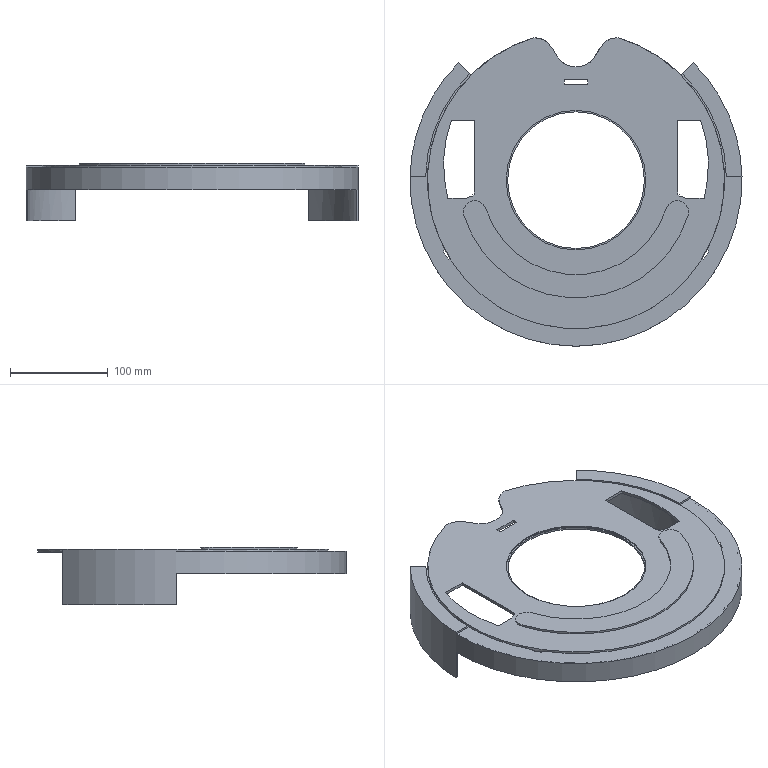Component | NX | OUTER_SHELL | 1 solid | 72 faces | volume 327418 mm3 | plane 49 | cylinder 21 | other 2 | commonest cylinder face diameters 308 x4 31.617 x2 271.2 x2 23.174 x2 23.617 x2 248.79 x1 304 x1 140 x1